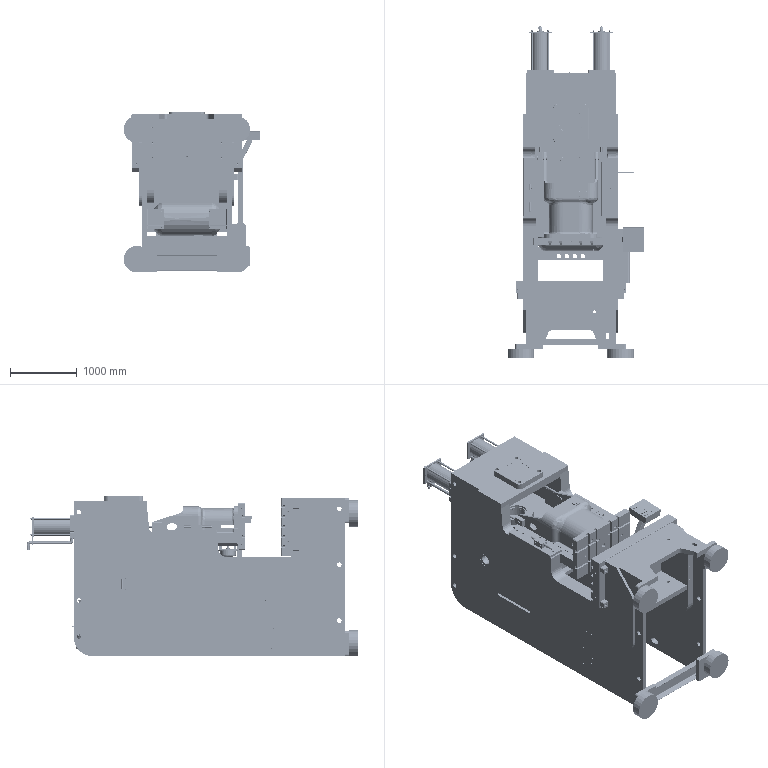Assembly | SolidWorks | mm | 141 component files | 205 solids | 8615 faces | box 2054 x 4987.81 x 2420 mm | volume 3140500679 mm3 | cylinder 3655 | plane 2654 | cone 1177 | spline 1129 | commonest cylinder face diameters 6.8 x207 4 x193 6 x189 9 x174 16 x130 20 x126 28 x116 17.5 x110
Bill of materials:
315InverterBracket() | 1 | Plain Carbon Steel | Thin L-shaped angle bracket of constant thickness, with two flanges meeting at a 90-degree bend. The longer flange has eight small holes, four at each end in 2x2 groups. The shorter flange has no visible holes. Outer corners are rounded.
400ShockAbsorbingPad | 4 | Plain Carbon Steel | Plain solid cylinder (disc or short round bar) with flat end faces. Its diameter is several times its length.
YC1-200-03-0202UpperWorkbench# | 1 | Plain Carbon Steel | Thick rectangular plate with T-slots machined into one face. The slots form a grid of four slots in one direction and two in the other. The plate has a larger central through-hole, several smaller through-holes, small holes in its edges and chamfered corners.
YC1-250-01-05RearCover | 1 | Plain Carbon Steel | Round flanged disc. A thin outer flange carries eight small holes evenly spaced around a bolt circle. A raised circular boss with a shallow circumferential groove in its side sits on the flange. A central through-bore passes through the part.
YC1-250-02-02CrankshaftBearingSeat | 1 | Plain Carbon Steel | Square flange block with rounded corners and a stepped cylindrical spigot on one side. It has a large central through-bore, four corner through-holes, two smaller diagonally placed holes, and a ring of very small holes or marks around a shallow counterbore.
YC1-250-02-05FrontCrankshaftBearing | 1 | Plain Carbon Steel | Thin-walled flanged sleeve or bushing: an open-ended cylindrical tube with a thin outward flange at one end. A faint line runs around the inside wall.
BearingGBNU2319E_RollingBearingsNU2319EGB283-94 | 1 | Plain Carbon Steel | Simplified model resembling a cylindrical roller bearing. Concentric inner and outer rings are separated by a ring of cylindrical rolling elements. The ring faces are flat and the edges are rounded.
YC1-250-02-03FrontDriveBearingSeat | 1 | Plain Carbon Steel | Round cover or end cap with a flange and a cylindrical spigot below it. The spigot has a circumferential groove and a chamfered end. The flange has six larger holes and two smaller holes. No central bore is visible.
YC1-250-02-23FrontDriveBearingSeatBearingGland | 1 | Plain Carbon Steel | Thin flat annular ring with a large central opening and six small holes evenly spaced around it.
YC1-250-02-20CrankshaftFrontEndAdjustmentCover | 1 | Plain Carbon Steel | Thick solid circular plate (blind-flange-like disc) with eight through-holes evenly spaced on a bolt circle. There is no central hole.
YC1-250-02-21CrankshaftEndCover | 1 | Plain Carbon Steel | Very thin flat circular disc with six small holes evenly spaced close to its outer edge. There is no central opening.
BearingGB-6309_RollingBearings6309GB276-94 | 2 | Plain Carbon Steel | Simplified model resembling a deep-groove ball bearing. Concentric inner and outer rings are separated by a single row of spherical balls. The ring faces are flat, the edges are rounded, and there are no visible seals or shields.
DigitalDisplayXSQ-1 | 1 | Plain Carbon Steel | Rectangular box-shaped body with a thin rectangular flange plate on top that sticks out past the body on all sides, plus one stepped cylindrical pin sticking out of the bottom, off-center.
Oil-impregnatedCopper | 1 | Plain Carbon Steel | Thin-walled cylindrical sleeve (ring) with many radial round holes through the wall, arranged in three rows around the circumference.
YC1-110-03-38LargeSprocketGland | 1 | Plain Carbon Steel | Flat circular disc with one central through-hole (washer-like).
YC1-160-03-22WormGland | 1 | Plain Carbon Steel | Round flanged ring: a flat circular base flange with a bolt-hole pattern, a raised cylindrical hub with an outer groove, and a stepped central bore.
YC1-160-03-32LargeSprocket | 1 | Plain Carbon Steel | Thin circular plate with a ring of six round holes and a two-step central hub with a keyed bore.
YC1-160-03-35Oil-impregnatedCopperSeat | 1 | Plain Carbon Steel | Thick-walled cylindrical bushing with a plain central bore and an outer ring groove near one end.
YC1-200-03-33SmallSprocket | 1 | Plain Carbon Steel | Flanged bushing: a wide, thin, chamfered circular flange on a smaller cylindrical body that has a neck under the flange, with a keyed central bore.
YC1-200-03-34DiscMotorSeat | 1 | Plain Carbon Steel | Flat square plate with a large central circular cutout, four corner slots and four small round holes.
YC1-200-03-39SmallSprocketGland | 1 | Plain Carbon Steel | Solid cylinder with a small central axial through-hole (spacer- or standoff-like).
YC1-250-03-01Slider | 1 | Plain Carbon Steel | Complex bracket or frame-like body: a rounded tunnel-shaped central section between side plates with mounting holes, sitting on a long rectangular base with rails.
YC1-250-03-04Worm | 1 | Plain Carbon Steel | Long stepped cylindrical shaft. Its largest diameter is a central section, and it steps down in several diameters toward both ends.
YC1-250-03-18BallHeadGland | 1 | Plain Carbon Steel | Flanged ring: a flat circular flange with a ring of holes, and a shorter cylindrical spigot on one side with a chamfered end, around a large central bore.
YC1-250-03-23HydraulicCylinderPressurePlate | 1 | Plain Carbon Steel | Long, narrow rectangular flat bar with small chamfers on the corners. It has two through-holes near each end, one large central through-hole and four smaller holes arranged around that central hole.
YC1-250-03-27BalancerConnectingPin | 2 | Plain Carbon Steel | Stepped, rotationally symmetric pin. A larger cylindrical body ends in a thin collar, then steps down to a smaller cylinder with a chamfered end. A small hole runs along the axis at the small end.
YC1-250-03-37Gland | 2 | Plain Carbon Steel | Flat circular disc with one small central through-hole. Compared with its diameter, the disc is moderately thick.
YC1-T-FCD-X8 | 1 | Plain Carbon Steel | Very thin, flat ring (annulus) with a large central opening, shaped like a shim or thin washer.
YPE1100S2-4Z | 1 | Plain Carbon Steel | Round, cup-shaped housing with a wider circular flange at one end. The flange has four through-holes equally spaced around it. A small cylindrical shaft sticks out from the centre of the flange face, and the closed end has rounded edges.
YC1-250-03-09RightGuideBushing | 2 | Plain Carbon Steel | Thin rectangular plate with sharp edges. It has four through-holes near the corners and two more holes along the horizontal centreline, set off toward one side.
YC1-250-03-12AdjustingPlate | 2 | Plain Carbon Steel | Thick rectangular block-plate. Each corner has one larger through-hole and one smaller hole beside it, the centre has a small hole, and one edge face has two small holes.
GBHexNutM20_GB_FASTENER_NUT_SNC1M16-N | 8 | Plain Carbon Steel | Long hexagonal prism with a large cylindrical bore through its length and chamfered ends. The overall shape resembles a long hex nut or coupling.
GBSpringWasherM20_GB_FASTENER_WASHER_SW16 | 8 | Plain Carbon Steel | Split ring with a rectangular cross-section and one narrow gap cut through it, on an angle.
Rc11-4Elbow | 4 | Plain Carbon Steel | Thin-walled tube with a 90-degree bend (elbow) and two straight legs at right angles, joined by a smooth bend.
Rc11-4StraightInternalConnection | 4 | Plain Carbon Steel | Hexagonal collar centred on a cylindrical sleeve that sticks out on both sides, with a cylindrical through-bore along the axis. The shape resembles a hex nipple or bushing.
YC1-250-04-01Base#16673 | 2 | Plain Carbon Steel | Rectangular plate with small chamfered corners. Each side edge has two open-ended U-shaped slots. The plate has one larger central hole and one smaller hole below it, and one face carries a shallow raised circular boss with a stepped or grooved rim.
YC1-250-04-02TopCover#16673(1) | 2 | Plain Carbon Steel | Flat rectangular plate with a large central through-hole, a shallow raised circular boss on one face concentric with the hole, and several smaller holes around it.
YC1-250-04-04CylinderBarrel#16673 | 2 | Plain Carbon Steel | Thin-walled, open-ended straight round tube.
YC1-250-04-05#16673Piston | 2 | Plain Carbon Steel | Disc-shaped grooved wheel with a small central bore and one groove around its rim.
YC1-250-04-06TieRodAxis#16673 | 2 | Plain Carbon Steel | Long, slender round shaft with short reduced-diameter stepped sections at both ends.
YC1-250-04-07TieRodSeat | 2 | Plain Carbon Steel | Rectangular block with an arch-shaped (U-shaped) slot cut through from one long edge, plus a small round through-hole beside the slot.
YC1-250-04-08Washer | 2 | Plain Carbon Steel | Flat annular washer-shaped ring with a large central hole.
YC1-250-04-09Cover | 2 | Plain Carbon Steel | Thin flat circular disc with two small through-holes placed opposite each other near the rim.
YC1-250-04-10Double-endedScrew#16673 | 8 | Plain Carbon Steel | Plain, solid, straight cylindrical rod.
YC1-250-04-11NipplePipe#16673 | 2 | Plain Carbon Steel | Straight round tube whose ends are slightly reduced or tapered.
YC1-250-04-12#16673PipeSeat | 2 | Plain Carbon Steel | Rectangular block with a round through-bore near one end and a thin straight gap running across the block through the bore's center line. It appears to be a split clamp-style block in two pieces.
YC1-250-04-13#16673Set | 8 | Plain Carbon Steel | Long, straight round tube with a moderately thick wall.
YC1-250-05-02EjectorRod | 1 | Plain Carbon Steel | Solid cylindrical pin with a chamfered or tapered lead-in at one end and a small circumferential groove or line near the other end.
YC1-250-05-03EjectorRodSeat | 1 | Plain Carbon Steel | Prismatic block with two chamfered corners on one end. A transverse through-bore has a narrow slit running from the bore to one face, giving a split-clamp shape. The top face has two larger through holes and a row of three smaller blind holes.
YC1-250-06-01AirTank | 1 | Plain Carbon Steel | Horizontal cylindrical vessel-like body with domed ends. It has two bent-plate support brackets along one side and several small cylindrical stubs on the shell.
YC1-250-06-03AirTankFixingSeat | 2 | Plain Carbon Steel | Bent sheet-metal angle bracket. A flat plate has a short folded flange along one edge and two tapered triangular gusset ribs. The edges have open-ended slots and slotted holes.
Coupling | 1 | Plain Carbon Steel | Short thick-walled cylindrical bushing with a central through-bore. The outside has three circumferential grooves and both outer edges are chamfered.
GB-61905_Rolling bearings 61905 GB 276-94 | 2 | Plain Carbon Steel | Rolling-element bearing-like ring assembly: outer ring, inner ring, and a full circle of spherical balls between them. No cage or shields are visible.
Sensor | 1 | Plain Carbon Steel | Cylindrical body with a raised coaxial pilot boss and a protruding plain cylindrical shaft on one end face. Three small holes sit on each end face, and a flat cutout is on the lower side.
YC1-250-09-05OutputShaft | 1 | Plain Carbon Steel | Long slender stepped cylindrical shaft. A small cross hole is near the larger end, and several successively smaller diameter steps are at the other end.
YC1-25-09-01Body | 1 | Plain Carbon Steel | Flanged housing with a circular flange that has a flat on one side and a bolt-hole pattern. A grooved tubular spigot extends above the flange. Below it is a tubular skirt with a large rectangular window, cross holes, and a side lug with a hole.
YC1-25-09-02Cam | 1 | Plain Carbon Steel | Thick D-shaped disc: a circle truncated by a straight chordal flat. It has a chamfered central through-hole and a small radial hole or pin feature visible inside the bore.
YC1-25-09-03Collar | 1 | Plain Carbon Steel | Plain cylindrical tube or sleeve with a large central bore, a uniform wall, and chamfered outer end edges.
YC1-25-09-04Cover | 1 | Plain Carbon Steel | Flat circular mounting plate truncated by a straight edge. It has a large central bore, an inner ring of four holes, an outer ring of six holes, and a raised annular step on one face.
YC1-25-01-08OilHoleCover | 1 | Plain Carbon Steel | Thin flat circular disc with two small through holes on opposite sides of the diameter.
YC1-250-02-06RearCrankshaftBearing | 1 | Plain Carbon Steel | Thin-walled short cylindrical sleeve/ring that is open at both ends, with a slightly larger lip at one end and a small chamfer at the other.
YC1-250-03-07RearGuideBushing | 4 | Plain Carbon Steel | Rectangular plate with one continuous serpentine groove on one face, four countersunk holes at the corners and one countersunk hole in the center.
YC1-250-03-08LeftGuideBushing | 2 | Plain Carbon Steel | Rectangular plate with a serpentine groove on one face, countersunk holes at the four corners and one countersunk hole in the center.
YC1-315-01-01Body#_Default_ByMachining | 1 | Plain Carbon Steel | Large, complex frame or housing built from plates, with a stepped top profile, side walls, internal cross members, large circular openings, rectangular windows and many small holes.
YC1-315-01-0402Workbench | 1 | Plain Carbon Steel | Thick rectangular block with a regular grid of through-holes on the large face, several larger and corner holes, and a row of stepped holes along one narrow edge.
TECOFixedSpeed30HP_4P | 1 | Plain Carbon Steel | Simplified cylindrical machine body with a protruding output shaft, a mounting flange or plate on the side, a lifting eye, feet at the base, a side terminal-box-like protrusion, and longitudinal ribs.
YC1-200-02-29AdjustingScrew | 4 | Plain Carbon Steel | Cylindrical sleeve with a central through-bore and a shorter hexagonal section at one end, similar in form to a standoff or spacer.
YC1-250-02-1801Pulley | 1 | Plain Carbon Steel | Multi-groove pulley-like wheel with five circumferential V-shaped grooves, a recessed face with a central hub, a keyed bore and two small holes in the web.
YC1-250-02-25MotorShaftEndCover | 1 | Plain Carbon Steel | Flat circular disc with one concentric central through-hole, similar in form to a washer.
YC1-315-02-28MotorMount | 1 | Plain Carbon Steel | Thin rectangular plate with four large corner holes, four pairs of small holes and a V-shaped notch in the middle of one short edge.
YC1-250-03-06FrontGuideBushing | 2 | Plain Carbon Steel | Long, thin flat bar with a row of small holes staggered along its length and clustered holes at each end.
YC1-315-03-10LeftPressurePlate | 1 | Plain Carbon Steel | Rectangular flat bar with a line of larger holes on its centerline, two smaller offset holes, a narrow transverse groove across the top face, and a stepped underside.
YC1-315-03-11RightPressurePlate | 1 | Plain Carbon Steel | Long, narrow, flat rectangular bar or plate with a row of through holes along its length and a thin line running across the top face.
80-315ControlPanel | 1 | Plain Carbon Steel | Solid rectangular block with an array of circular holes and shallow round recesses on the top face, plus a thin L-shaped line marking.
80-315ElectricBox | 1 | Plain Carbon Steel | Box-shaped, thin-walled enclosure or cover with rounded long edges, a rectangular opening on the top face, and protruding mounting tabs on two opposite sides.
YC1-160BoxBaffleT | 1 | Plain Carbon Steel | Thin, flat square frame-shaped plate with a large central square opening that has rounded corners.
YC1-160OperationStationBaffleT | 1 | Plain Carbon Steel | Thin rectangular plate with an off-center rectangular through-opening and four small corner holes.
YC1-315OperationStationConnectingArmT_Default_ByMachining | 1 | Plain Carbon Steel | Hollow square or rectangular tube with a jog bend (offset) near one end, so the short end section is parallel to but offset from the main straight length.
YC1-315SmallBracketT | 1 | Plain Carbon Steel | Bent, sheet-like hat-section bracket: a raised center channel with two coplanar outer flanges, each flange having two obround slots.
Mates: